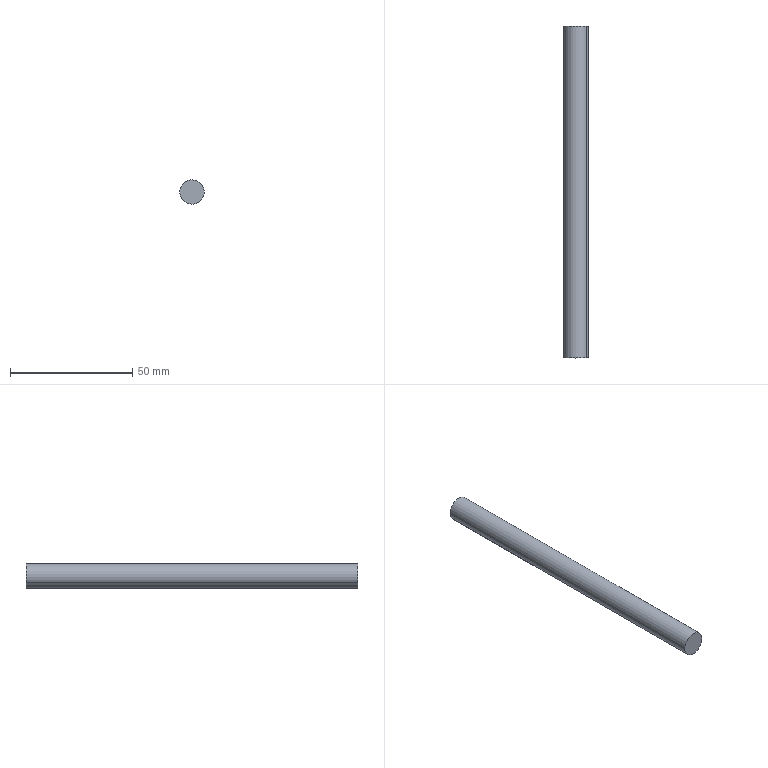Component | SolidWorks | Axis1-1 | 1 solid | 8 faces | box 10 x 136 x 10 mm | volume 10377 mm3 | cylinder 4 | cone 2 | plane 2 | commonest cylinder face diameters 5 x2 10 x2
build123d program:
from build123d import *

# Parameters (mm, degrees)
SKETCH1_R             = 5
BOSS_EXTRUDE1_DEPTH   = 136
M6_TAPPED_HOLE1_D     = 5
M6_TAPPED_HOLE1_DEPTH = 15
M6_TAPPED_HOLE1_TIP   = 1.502


with BuildPart() as part:
    # Sketch1 → Boss-Extrude1 (new body)
    with BuildSketch(Plane.XY):
        Circle(SKETCH1_R)
    extrude(amount=BOSS_EXTRUDE1_DEPTH)

    # M6 Tapped Hole1
    with Locations(Plane(origin=(0, 0, 0), x_dir=(-1, 0, 0), z_dir=(0, 0, -1))):
        with Locations((0, 0)):
            Hole(M6_TAPPED_HOLE1_D / 2, depth=M6_TAPPED_HOLE1_DEPTH)
            with Locations((0, 0, -(M6_TAPPED_HOLE1_DEPTH + M6_TAPPED_HOLE1_TIP / 2))):  # 118° drill point
                Cone(0, M6_TAPPED_HOLE1_D / 2, M6_TAPPED_HOLE1_TIP, mode=Mode.SUBTRACT)


solid = part.part

# Placed as in the assembly
solid = solid.moved(Location((-60.547, -21.54, 258), (90, 0, 0)))
STEP:
#1=COLOUR_RGB('',0.7922,0.8196,0.9333);
#2=FILL_AREA_STYLE_COLOUR('',#1);
#3=FILL_AREA_STYLE('',(#2));
#4=SURFACE_STYLE_FILL_AREA(#3);
#5=SURFACE_SIDE_STYLE('',(#4));
#6=SURFACE_STYLE_USAGE(.BOTH.,#5);
#7=PRESENTATION_STYLE_ASSIGNMENT((#6));
#8=CARTESIAN_POINT('',(-2.301,-1.439,10.211));
#9=VERTEX_POINT('',#8);
#10=CARTESIAN_POINT('',(-2.466,-1.439,10.104));
#11=VERTEX_POINT('',#10);
#12=CARTESIAN_POINT('',(-2.384,-1.439,10.157));
#13=DIRECTION('',(-0.,1.,-0.));
#14=DIRECTION('',(-0.8372,0.,-0.5469));
#15=AXIS2_PLACEMENT_3D('',#12,#13,#14);
#16=CIRCLE('',#15,0.09843);
#17=EDGE_CURVE('',#9,#11,#16,.T.);
#18=ORIENTED_EDGE('',*,*,#17,.F.);
#19=CARTESIAN_POINT('',(-2.301,-0.848,10.211));
#20=VERTEX_POINT('',#19);
#21=CARTESIAN_POINT('',(-2.301,-0.848,10.211));
#22=DIRECTION('',(-0.,1.,-0.));
#23=VECTOR('',#22,39.37);
#24=LINE('',#21,#23);
#25=EDGE_CURVE('',#9,#20,#24,.T.);
#26=ORIENTED_EDGE('',*,*,#25,.T.);
#27=CARTESIAN_POINT('',(-2.466,-0.848,10.104));
#28=VERTEX_POINT('',#27);
#29=CARTESIAN_POINT('',(-2.384,-0.848,10.157));
#30=DIRECTION('',(-0.,1.,-0.));
#31=DIRECTION('',(-0.8372,0.,-0.5469));
#32=AXIS2_PLACEMENT_3D('',#29,#30,#31);
#33=CIRCLE('',#32,0.09843);
#34=EDGE_CURVE('',#20,#28,#33,.T.);
#35=ORIENTED_EDGE('',*,*,#34,.T.);
#36=CARTESIAN_POINT('',(-2.466,-0.848,10.104));
#37=DIRECTION('',(-0.,1.,-0.));
#38=VECTOR('',#37,39.37);
#39=LINE('',#36,#38);
#40=EDGE_CURVE('',#11,#28,#39,.T.);
#41=ORIENTED_EDGE('',*,*,#40,.F.);
#42=EDGE_LOOP('',(#18,#26,#35,#41));
#43=FACE_OUTER_BOUND('',#42,.T.);
#44=CARTESIAN_POINT('',(-2.384,-0.848,10.157));
#45=DIRECTION('',(-0.,1.,-0.));
#46=DIRECTION('',(-0.8372,0.,-0.5469));
#47=AXIS2_PLACEMENT_3D('',#44,#45,#46);
#48=CYLINDRICAL_SURFACE('',#47,0.09843);
#49=ADVANCED_FACE('',(#43),#48,.F.);
#50=CARTESIAN_POINT('',(-2.384,-1.498,10.157));
#51=VERTEX_POINT('',#50);
#52=CARTESIAN_POINT('',(-2.466,-1.439,10.104));
#53=DIRECTION('',(-0.7176,0.515,-0.4688));
#54=VECTOR('',#53,39.37);
#55=LINE('',#52,#54);
#56=EDGE_CURVE('',#51,#11,#55,.T.);
#57=ORIENTED_EDGE('',*,*,#56,.F.);
#58=CARTESIAN_POINT('',(-2.301,-1.439,10.211));
#59=DIRECTION('',(0.7176,0.515,0.4688));
#60=VECTOR('',#59,39.37);
#61=LINE('',#58,#60);
#62=EDGE_CURVE('',#51,#9,#61,.T.);
#63=ORIENTED_EDGE('',*,*,#62,.T.);
#64=ORIENTED_EDGE('',*,*,#17,.T.);
#65=EDGE_LOOP('',(#57,#63,#64));
#66=FACE_OUTER_BOUND('',#65,.T.);
#67=CARTESIAN_POINT('',(-2.384,-1.439,10.157));
#68=DIRECTION('',(-0.,1.,-0.));
#69=DIRECTION('',(-0.8372,0.,-0.5469));
#70=AXIS2_PLACEMENT_3D('',#67,#68,#69);
#71=CONICAL_SURFACE('',#70,0.09843,1.03);
#72=ADVANCED_FACE('',(#66),#71,.F.);
#73=CARTESIAN_POINT('',(-2.219,-6.202,10.265));
#74=VERTEX_POINT('',#73);
#75=CARTESIAN_POINT('',(-2.549,-6.202,10.05));
#76=VERTEX_POINT('',#75);
#77=CARTESIAN_POINT('',(-2.384,-6.202,10.157));
#78=DIRECTION('',(0.,-1.,0.));
#79=DIRECTION('',(0.8372,0.,0.5469));
#80=AXIS2_PLACEMENT_3D('',#77,#78,#79);
#81=CIRCLE('',#80,0.1969);
#82=EDGE_CURVE('',#74,#76,#81,.T.);
#83=ORIENTED_EDGE('',*,*,#82,.F.);
#84=CARTESIAN_POINT('',(-2.219,-0.848,10.265));
#85=VERTEX_POINT('',#84);
#86=CARTESIAN_POINT('',(-2.219,-6.202,10.265));
#87=DIRECTION('',(-0.,1.,-0.));
#88=VECTOR('',#87,39.37);
#89=LINE('',#86,#88);
#90=EDGE_CURVE('',#74,#85,#89,.T.);
#91=ORIENTED_EDGE('',*,*,#90,.T.);
#92=CARTESIAN_POINT('',(-2.549,-0.848,10.05));
#93=VERTEX_POINT('',#92);
#94=CARTESIAN_POINT('',(-2.384,-0.848,10.157));
#95=DIRECTION('',(0.,-1.,0.));
#96=DIRECTION('',(0.8372,0.,0.5469));
#97=AXIS2_PLACEMENT_3D('',#94,#95,#96);
#98=CIRCLE('',#97,0.1969);
#99=EDGE_CURVE('',#85,#93,#98,.T.);
#100=ORIENTED_EDGE('',*,*,#99,.T.);
#101=CARTESIAN_POINT('',(-2.549,-6.202,10.05));
#102=DIRECTION('',(-0.,1.,-0.));
#103=VECTOR('',#102,39.37);
#104=LINE('',#101,#103);
#105=EDGE_CURVE('',#76,#93,#104,.T.);
#106=ORIENTED_EDGE('',*,*,#105,.F.);
#107=EDGE_LOOP('',(#83,#91,#100,#106));
#108=FACE_OUTER_BOUND('',#107,.T.);
#109=CARTESIAN_POINT('',(-2.384,-6.202,10.157));
#110=DIRECTION('',(-0.,1.,-0.));
#111=DIRECTION('',(-0.8372,0.,-0.5469));
#112=AXIS2_PLACEMENT_3D('',#109,#110,#111);
#113=CYLINDRICAL_SURFACE('',#112,0.1969);
#114=ADVANCED_FACE('',(#108),#113,.T.);
#115=ORIENTED_EDGE('',*,*,#90,.F.);
#116=CARTESIAN_POINT('',(-2.384,-6.202,10.157));
#117=DIRECTION('',(0.,-1.,0.));
#118=DIRECTION('',(0.8372,0.,0.5469));
#119=AXIS2_PLACEMENT_3D('',#116,#117,#118);
#120=CIRCLE('',#119,0.1969);
#121=EDGE_CURVE('',#76,#74,#120,.T.);
#122=ORIENTED_EDGE('',*,*,#121,.F.);
#123=ORIENTED_EDGE('',*,*,#105,.T.);
#124=CARTESIAN_POINT('',(-2.384,-0.848,10.157));
#125=DIRECTION('',(0.,-1.,0.));
#126=DIRECTION('',(0.8372,0.,0.5469));
#127=AXIS2_PLACEMENT_3D('',#124,#125,#126);
#128=CIRCLE('',#127,0.1969);
#129=EDGE_CURVE('',#93,#85,#128,.T.);
#130=ORIENTED_EDGE('',*,*,#129,.T.);
#131=EDGE_LOOP('',(#115,#122,#123,#130));
#132=FACE_OUTER_BOUND('',#131,.T.);
#133=CARTESIAN_POINT('',(-2.384,-6.202,10.157));
#134=DIRECTION('',(-0.,1.,-0.));
#135=DIRECTION('',(-0.8372,0.,-0.5469));
#136=AXIS2_PLACEMENT_3D('',#133,#134,#135);
#137=CYLINDRICAL_SURFACE('',#136,0.1969);
#138=ADVANCED_FACE('',(#132),#137,.T.);
#139=ORIENTED_EDGE('',*,*,#121,.T.);
#140=ORIENTED_EDGE('',*,*,#82,.T.);
#141=EDGE_LOOP('',(#139,#140));
#142=FACE_OUTER_BOUND('',#141,.T.);
#143=CARTESIAN_POINT('',(-2.384,-6.202,10.157));
#144=DIRECTION('',(0.,-1.,0.));
#145=DIRECTION('',(0.8372,0.,0.5469));
#146=AXIS2_PLACEMENT_3D('',#143,#144,#145);
#147=PLANE('',#146);
#148=ADVANCED_FACE('',(#142),#147,.T.);
#149=CARTESIAN_POINT('',(-2.384,-0.848,10.157));
#150=DIRECTION('',(-0.,1.,-0.));
#151=DIRECTION('',(-0.8372,0.,-0.5469));
#152=AXIS2_PLACEMENT_3D('',#149,#150,#151);
#153=CIRCLE('',#152,0.09843);
#154=EDGE_CURVE('',#28,#20,#153,.T.);
#155=ORIENTED_EDGE('',*,*,#154,.F.);
#156=ORIENTED_EDGE('',*,*,#34,.F.);
#157=EDGE_LOOP('',(#155,#156));
#158=FACE_BOUND('',#157,.T.);
#159=ORIENTED_EDGE('',*,*,#129,.F.);
#160=ORIENTED_EDGE('',*,*,#99,.F.);
#161=EDGE_LOOP('',(#159,#160));
#162=FACE_OUTER_BOUND('',#161,.T.);
#163=CARTESIAN_POINT('',(-2.384,-0.848,10.157));
#164=DIRECTION('',(0.,-1.,0.));
#165=DIRECTION('',(0.8372,0.,0.5469));
#166=AXIS2_PLACEMENT_3D('',#163,#164,#165);
#167=PLANE('',#166);
#168=ADVANCED_FACE('',(#158,#162),#167,.F.);
#169=ORIENTED_EDGE('',*,*,#62,.F.);
#170=ORIENTED_EDGE('',*,*,#56,.T.);
#171=CARTESIAN_POINT('',(-2.384,-1.439,10.157));
#172=DIRECTION('',(-0.,1.,-0.));
#173=DIRECTION('',(-0.8372,0.,-0.5469));
#174=AXIS2_PLACEMENT_3D('',#171,#172,#173);
#175=CIRCLE('',#174,0.09843);
#176=EDGE_CURVE('',#11,#9,#175,.T.);
#177=ORIENTED_EDGE('',*,*,#176,.T.);
#178=EDGE_LOOP('',(#169,#170,#177));
#179=FACE_OUTER_BOUND('',#178,.T.);
#180=CARTESIAN_POINT('',(-2.384,-1.439,10.157));
#181=DIRECTION('',(-0.,1.,-0.));
#182=DIRECTION('',(-0.8372,0.,-0.5469));
#183=AXIS2_PLACEMENT_3D('',#180,#181,#182);
#184=CONICAL_SURFACE('',#183,0.09843,1.03);
#185=ADVANCED_FACE('',(#179),#184,.F.);
#186=ORIENTED_EDGE('',*,*,#25,.F.);
#187=ORIENTED_EDGE('',*,*,#176,.F.);
#188=ORIENTED_EDGE('',*,*,#40,.T.);
#189=ORIENTED_EDGE('',*,*,#154,.T.);
#190=EDGE_LOOP('',(#186,#187,#188,#189));
#191=FACE_OUTER_BOUND('',#190,.T.);
#192=CARTESIAN_POINT('',(-2.384,-0.848,10.157));
#193=DIRECTION('',(-0.,1.,-0.));
#194=DIRECTION('',(-0.8372,0.,-0.5469));
#195=AXIS2_PLACEMENT_3D('',#192,#193,#194);
#196=CYLINDRICAL_SURFACE('',#195,0.09843);
#197=ADVANCED_FACE('',(#191),#196,.F.);
#198=CLOSED_SHELL('',(#49,#72,#114,#138,#148,#168,#185,#197));
#199=MANIFOLD_SOLID_BREP('',#198);
#200=STYLED_ITEM('',(#7),#199);
#201=(LENGTH_UNIT()NAMED_UNIT(*)SI_UNIT($,.METRE.));
#202=LENGTH_MEASURE_WITH_UNIT(LENGTH_MEASURE(0.0254),#201);
#203=DIMENSIONAL_EXPONENTS(1.,0.,0.,0.,0.,0.,0.);
#204=(CONVERSION_BASED_UNIT('',#202)LENGTH_UNIT()NAMED_UNIT(#203));
#205=UNCERTAINTY_MEASURE_WITH_UNIT(LENGTH_MEASURE(0.00001),#204,'','');
#206=(NAMED_UNIT(*)PLANE_ANGLE_UNIT()SI_UNIT($,.RADIAN.));
#207=(NAMED_UNIT(*)SI_UNIT($,.STERADIAN.)SOLID_ANGLE_UNIT());
#208=(GEOMETRIC_REPRESENTATION_CONTEXT(3)GLOBAL_UNCERTAINTY_ASSIGNED_CONTEXT((#205))GLOBAL_UNIT_ASSIGNED_CONTEXT((#204,#206,#207))REPRESENTATION_CONTEXT('',''));
#209=MECHANICAL_DESIGN_GEOMETRIC_PRESENTATION_REPRESENTATION('',(#200),#208);
#210=PRESENTATION_LAYER_ASSIGNMENT('','',(#200));
#211=CARTESIAN_POINT('',(0.,0.,0.));
#212=DIRECTION('',(0.,0.,1.));
#213=DIRECTION('',(1.,0.,0.));
#214=AXIS2_PLACEMENT_3D('',#211,#212,#213);
#215=(LENGTH_UNIT()NAMED_UNIT(*)SI_UNIT($,.METRE.));
#216=LENGTH_MEASURE_WITH_UNIT(LENGTH_MEASURE(0.0254),#215);
#217=DIMENSIONAL_EXPONENTS(1.,0.,0.,0.,0.,0.,0.);
#218=(CONVERSION_BASED_UNIT('',#216)LENGTH_UNIT()NAMED_UNIT(#217));
#219=UNCERTAINTY_MEASURE_WITH_UNIT(LENGTH_MEASURE(0.00001),#218,'','');
#220=(NAMED_UNIT(*)PLANE_ANGLE_UNIT()SI_UNIT($,.RADIAN.));
#221=(NAMED_UNIT(*)SI_UNIT($,.STERADIAN.)SOLID_ANGLE_UNIT());
#222=(GEOMETRIC_REPRESENTATION_CONTEXT(3)GLOBAL_UNCERTAINTY_ASSIGNED_CONTEXT((#219))GLOBAL_UNIT_ASSIGNED_CONTEXT((#218,#220,#221))REPRESENTATION_CONTEXT('',''));
#223=ADVANCED_BREP_SHAPE_REPRESENTATION('',(#199,#214),#222);